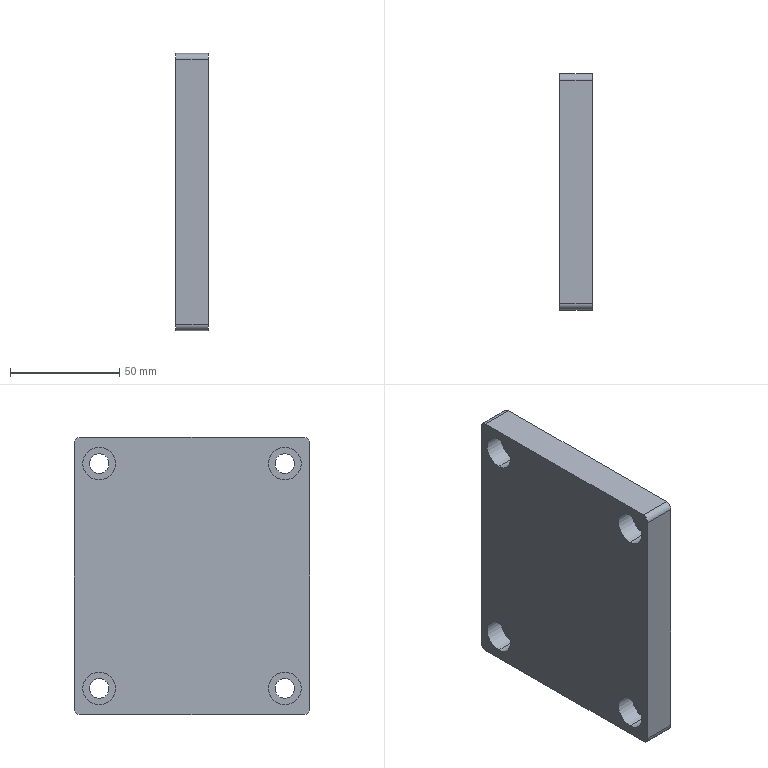Component | SolidWorks | 19-1 | 1 solid | 39 faces | box 15 x 108 x 127 mm | volume 171943 mm3 | cylinder 24 | plane 15 | commonest cylinder face diameters 15 x8 9 x8 6 x8
build123d program:
from build123d import *

# Parameters (mm, degrees)
SKETCH1_W           = 108
SKETCH1_H           = 127
BOSS_EXTRUDE1_DEPTH = 15
SKETCH2_W           = 62
SKETCH2_H           = 85
CUT_EXTRUDE1_DEPTH  = 5
FILLET1_R           = 3
FILLET2_R           = 3
HOLE2_D             = 9
HOLE2_DEPTH         = 99.955
HOLE2_CBORE_D       = 15
HOLE2_CBORE_DEPTH   = 9


with BuildPart() as part:
    # Sketch1 → Boss-Extrude1 (new body)
    with BuildSketch(Plane(origin=(0, 0, 0), x_dir=(1, 0, 0), z_dir=(0, 1, 0))):
        Rectangle(SKETCH1_W, SKETCH1_H)
    extrude(amount=BOSS_EXTRUDE1_DEPTH)

    # Sketch2 → Cut-Extrude1 (cut)
    with BuildSketch(Plane(origin=(0, 15, 0), x_dir=(1, 0, 0), z_dir=(0, 1, 0))):
        Rectangle(SKETCH2_W, SKETCH2_H)
    extrude(amount=-CUT_EXTRUDE1_DEPTH, mode=Mode.SUBTRACT)

    # Fillet1
    fillet1_edges = [part.edges().sort_by_distance(p)[0] for p in [
        (31, 10, 0),
        (0, 10, 42.5),
        (-31, 10, 0),
        (0, 10, -42.5),
    ]]
    fillet(fillet1_edges, radius=FILLET1_R)

    # Fillet2
    fillet2_edges = [part.edges().sort_by_distance(p)[0] for p in [
        (54, 7.5, 63.5),
        (-54, 7.5, 63.5),
        (-54, 7.5, -63.5),
        (54, 7.5, -63.5),
    ]]
    fillet(fillet2_edges, radius=FILLET2_R)

    # Hole2
    with Locations(Plane(origin=(0, 0, 0), x_dir=(-1, 0, 0), z_dir=(0, -1, 0))):
        with Locations((-42.5, 51.5), (42.5, 51.5), (42.5, -51.5), (-42.5, -51.5)):
            CounterBoreHole(HOLE2_D / 2, HOLE2_CBORE_D / 2, HOLE2_CBORE_DEPTH, depth=HOLE2_DEPTH)


solid = part.part

# Placed as in the assembly
solid = solid.moved(Location((-101, -47, 0), (0, 0, -90)))